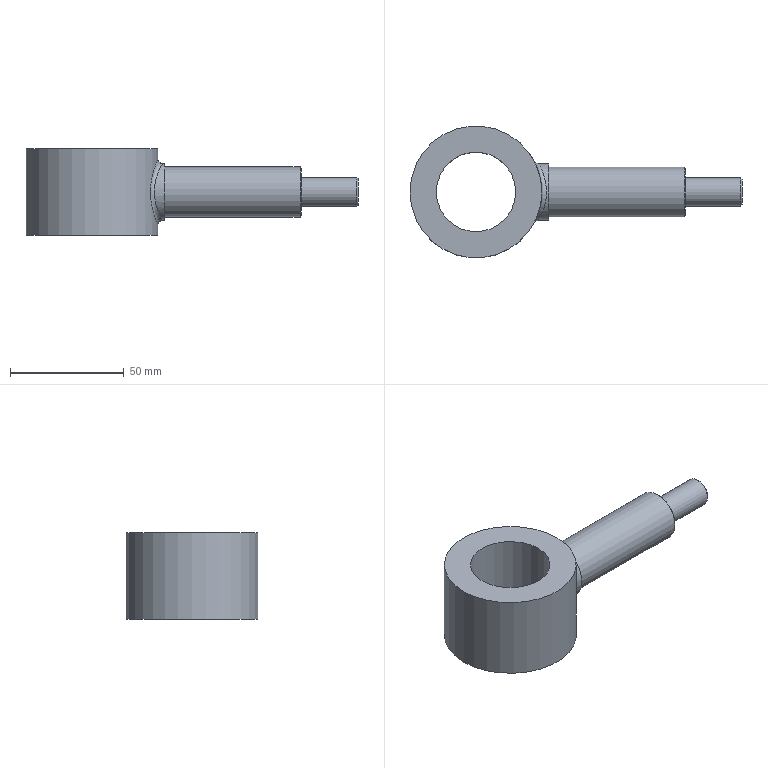Component | NX | WORKPIECE | 1 solid | 13 faces | volume 91555 mm3 | cylinder 5 | plane 5 | cone 2 | spline 1 | commonest cylinder face diameters 58 x1 25 x1 12.5 x1 22 x1 35 x1